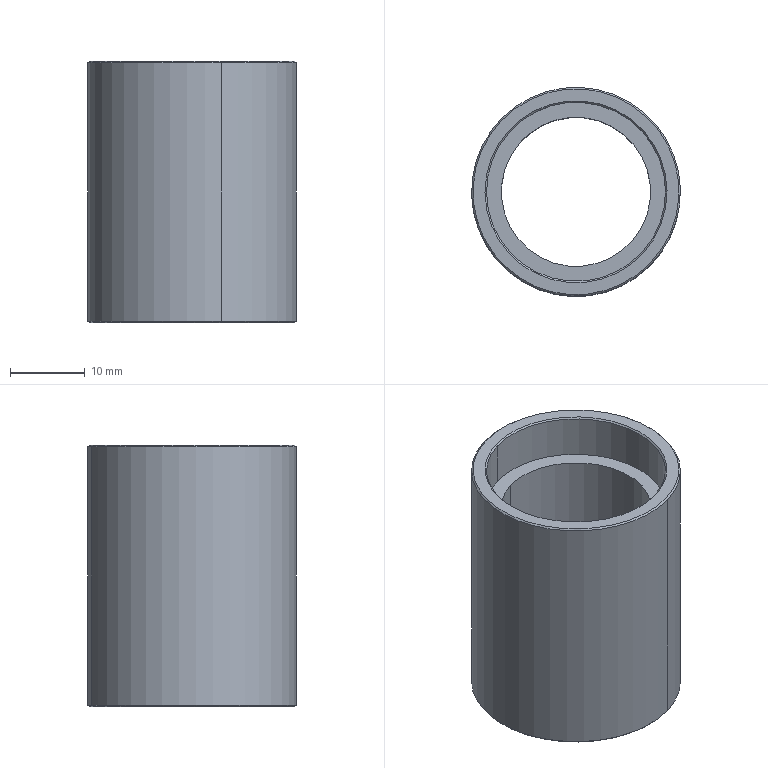Component | SolidWorks | GluePaperFeedingPressureRollerAssembly-1_YX-04-112GluePaperFeedingBearingFixingSleeve-1 | 1 solid | 20 faces | box 28 x 28 x 35 mm | volume 8890 mm3 | cylinder 8 | cone 8 | plane 4 | commonest cylinder face diameters 24 x4 20 x2 28 x2 | material 45#Steel
build123d program:
from build123d import *


with BuildPart() as part:
    # Sketch1 → Revolve1 (revolve)
    with BuildSketch(Plane.XY, mode=Mode.PRIVATE) as revolve1_sk:
        Polygon((-11.5, 12), (-11.5, 10), (11.5, 10), (11.5, 12), (17.3, 12), (17.5, 12.2), (17.5, 13.8), (17.3, 14), (-17.3, 14), (-17.5, 13.8), (-17.5, 12.2), (-17.3, 12), align=None)
    revolve(revolve1_sk.sketch.rotate(Axis((-17.5, 0, 0), (1, 0, 0)), 270), axis=Axis((-17.5, 0, 0), (1, 0, 0)))


solid = part.part

# Placed as in the assembly
solid = solid.moved(Location((-23.397, 0.262, 136.5), (0, 90, 0)))
STEP:
#1=COLOUR_RGB('',0.7922,0.8196,0.9333);
#2=FILL_AREA_STYLE_COLOUR('',#1);
#3=FILL_AREA_STYLE('',(#2));
#4=SURFACE_STYLE_FILL_AREA(#3);
#5=SURFACE_SIDE_STYLE('',(#4));
#6=SURFACE_STYLE_USAGE(.BOTH.,#5);
#7=PRESENTATION_STYLE_ASSIGNMENT((#6));
#8=CARTESIAN_POINT('',(-0.81,-0.3674,5.827));
#9=VERTEX_POINT('',#8);
#10=CARTESIAN_POINT('',(-1.032,0.388,5.827));
#11=VERTEX_POINT('',#10);
#12=CARTESIAN_POINT('',(-0.9212,0.01031,5.827));
#13=DIRECTION('',(-0.,0.,-1.));
#14=DIRECTION('',(-0.2824,0.9593,0.));
#15=AXIS2_PLACEMENT_3D('',#12,#13,#14);
#16=CIRCLE('',#15,0.3937);
#17=EDGE_CURVE('',#9,#11,#16,.T.);
#18=ORIENTED_EDGE('',*,*,#17,.F.);
#19=CARTESIAN_POINT('',(-0.81,-0.3674,4.921));
#20=VERTEX_POINT('',#19);
#21=CARTESIAN_POINT('',(-0.81,-0.3674,6.063));
#22=DIRECTION('',(-0.,0.,-1.));
#23=VECTOR('',#22,39.37);
#24=LINE('',#21,#23);
#25=EDGE_CURVE('',#9,#20,#24,.T.);
#26=ORIENTED_EDGE('',*,*,#25,.T.);
#27=CARTESIAN_POINT('',(-1.032,0.388,4.921));
#28=VERTEX_POINT('',#27);
#29=CARTESIAN_POINT('',(-0.9212,0.01031,4.921));
#30=DIRECTION('',(-0.,0.,-1.));
#31=DIRECTION('',(-0.2824,0.9593,0.));
#32=AXIS2_PLACEMENT_3D('',#29,#30,#31);
#33=CIRCLE('',#32,0.3937);
#34=EDGE_CURVE('',#20,#28,#33,.T.);
#35=ORIENTED_EDGE('',*,*,#34,.T.);
#36=CARTESIAN_POINT('',(-1.032,0.388,6.063));
#37=DIRECTION('',(-0.,0.,-1.));
#38=VECTOR('',#37,39.37);
#39=LINE('',#36,#38);
#40=EDGE_CURVE('',#11,#28,#39,.T.);
#41=ORIENTED_EDGE('',*,*,#40,.F.);
#42=EDGE_LOOP('',(#18,#26,#35,#41));
#43=FACE_OUTER_BOUND('',#42,.T.);
#44=CARTESIAN_POINT('',(-0.9212,0.01031,6.063));
#45=DIRECTION('',(-0.,0.,-1.));
#46=DIRECTION('',(-0.2824,0.9593,0.));
#47=AXIS2_PLACEMENT_3D('',#44,#45,#46);
#48=CYLINDRICAL_SURFACE('',#47,0.3937);
#49=ADVANCED_FACE('',(#43),#48,.F.);
#50=CARTESIAN_POINT('',(-0.7877,-0.4429,4.921));
#51=VERTEX_POINT('',#50);
#52=CARTESIAN_POINT('',(-1.055,0.4635,4.921));
#53=VERTEX_POINT('',#52);
#54=CARTESIAN_POINT('',(-0.9212,0.01031,4.921));
#55=DIRECTION('',(-0.,0.,-1.));
#56=DIRECTION('',(-0.2824,0.9593,0.));
#57=AXIS2_PLACEMENT_3D('',#54,#55,#56);
#58=CIRCLE('',#57,0.4724);
#59=EDGE_CURVE('',#51,#53,#58,.T.);
#60=ORIENTED_EDGE('',*,*,#59,.F.);
#61=CARTESIAN_POINT('',(-0.7877,-0.4429,4.693));
#62=VERTEX_POINT('',#61);
#63=CARTESIAN_POINT('',(-0.7877,-0.4429,6.063));
#64=DIRECTION('',(-0.,0.,-1.));
#65=VECTOR('',#64,39.37);
#66=LINE('',#63,#65);
#67=EDGE_CURVE('',#51,#62,#66,.T.);
#68=ORIENTED_EDGE('',*,*,#67,.T.);
#69=CARTESIAN_POINT('',(-1.055,0.4635,4.693));
#70=VERTEX_POINT('',#69);
#71=CARTESIAN_POINT('',(-0.9212,0.01031,4.693));
#72=DIRECTION('',(-0.,0.,-1.));
#73=DIRECTION('',(-0.2824,0.9593,0.));
#74=AXIS2_PLACEMENT_3D('',#71,#72,#73);
#75=CIRCLE('',#74,0.4724);
#76=EDGE_CURVE('',#62,#70,#75,.T.);
#77=ORIENTED_EDGE('',*,*,#76,.T.);
#78=CARTESIAN_POINT('',(-1.055,0.4635,6.063));
#79=DIRECTION('',(-0.,0.,-1.));
#80=VECTOR('',#79,39.37);
#81=LINE('',#78,#80);
#82=EDGE_CURVE('',#53,#70,#81,.T.);
#83=ORIENTED_EDGE('',*,*,#82,.F.);
#84=EDGE_LOOP('',(#60,#68,#77,#83));
#85=FACE_OUTER_BOUND('',#84,.T.);
#86=CARTESIAN_POINT('',(-0.9212,0.01031,6.063));
#87=DIRECTION('',(-0.,0.,-1.));
#88=DIRECTION('',(-0.2824,0.9593,0.));
#89=AXIS2_PLACEMENT_3D('',#86,#87,#88);
#90=CYLINDRICAL_SURFACE('',#89,0.4724);
#91=ADVANCED_FACE('',(#85),#90,.F.);
#92=ORIENTED_EDGE('',*,*,#76,.F.);
#93=CARTESIAN_POINT('',(-0.7855,-0.4505,4.685));
#94=VERTEX_POINT('',#93);
#95=CARTESIAN_POINT('',(-0.7877,-0.4429,4.693));
#96=DIRECTION('',(0.1997,-0.6783,-0.7071));
#97=VECTOR('',#96,39.37);
#98=LINE('',#95,#97);
#99=EDGE_CURVE('',#62,#94,#98,.T.);
#100=ORIENTED_EDGE('',*,*,#99,.T.);
#101=CARTESIAN_POINT('',(-1.057,0.4711,4.685));
#102=VERTEX_POINT('',#101);
#103=CARTESIAN_POINT('',(-0.9212,0.01031,4.685));
#104=DIRECTION('',(-0.,0.,-1.));
#105=DIRECTION('',(-0.2824,0.9593,0.));
#106=AXIS2_PLACEMENT_3D('',#103,#104,#105);
#107=CIRCLE('',#106,0.4803);
#108=EDGE_CURVE('',#94,#102,#107,.T.);
#109=ORIENTED_EDGE('',*,*,#108,.T.);
#110=CARTESIAN_POINT('',(-1.055,0.4635,4.693));
#111=DIRECTION('',(-0.1997,0.6783,-0.7071));
#112=VECTOR('',#111,39.37);
#113=LINE('',#110,#112);
#114=EDGE_CURVE('',#70,#102,#113,.T.);
#115=ORIENTED_EDGE('',*,*,#114,.F.);
#116=EDGE_LOOP('',(#92,#100,#109,#115));
#117=FACE_OUTER_BOUND('',#116,.T.);
#118=CARTESIAN_POINT('',(-0.9212,0.01031,4.693));
#119=DIRECTION('',(-0.,0.,-1.));
#120=DIRECTION('',(-0.2824,0.9593,0.));
#121=AXIS2_PLACEMENT_3D('',#118,#119,#120);
#122=CONICAL_SURFACE('',#121,0.4724,0.7854);
#123=ADVANCED_FACE('',(#117),#122,.F.);
#124=CARTESIAN_POINT('',(-1.075,0.5315,4.685));
#125=VERTEX_POINT('',#124);
#126=CARTESIAN_POINT('',(-0.7677,-0.5109,4.685));
#127=VERTEX_POINT('',#126);
#128=CARTESIAN_POINT('',(-0.9212,0.01031,4.685));
#129=DIRECTION('',(-0.,0.,-1.));
#130=DIRECTION('',(-0.2824,0.9593,0.));
#131=AXIS2_PLACEMENT_3D('',#128,#129,#130);
#132=CIRCLE('',#131,0.5433);
#133=EDGE_CURVE('',#125,#127,#132,.T.);
#134=ORIENTED_EDGE('',*,*,#133,.F.);
#135=CARTESIAN_POINT('',(-1.077,0.5391,4.693));
#136=VERTEX_POINT('',#135);
#137=CARTESIAN_POINT('',(-1.075,0.5315,4.685));
#138=DIRECTION('',(-0.1997,0.6783,0.7071));
#139=VECTOR('',#138,39.37);
#140=LINE('',#137,#139);
#141=EDGE_CURVE('',#125,#136,#140,.T.);
#142=ORIENTED_EDGE('',*,*,#141,.T.);
#143=CARTESIAN_POINT('',(-0.7655,-0.5184,4.693));
#144=VERTEX_POINT('',#143);
#145=CARTESIAN_POINT('',(-0.9212,0.01031,4.693));
#146=DIRECTION('',(-0.,0.,-1.));
#147=DIRECTION('',(-0.2824,0.9593,0.));
#148=AXIS2_PLACEMENT_3D('',#145,#146,#147);
#149=CIRCLE('',#148,0.5512);
#150=EDGE_CURVE('',#136,#144,#149,.T.);
#151=ORIENTED_EDGE('',*,*,#150,.T.);
#152=CARTESIAN_POINT('',(-0.7677,-0.5109,4.685));
#153=DIRECTION('',(0.1997,-0.6783,0.7071));
#154=VECTOR('',#153,39.37);
#155=LINE('',#152,#154);
#156=EDGE_CURVE('',#127,#144,#155,.T.);
#157=ORIENTED_EDGE('',*,*,#156,.F.);
#158=EDGE_LOOP('',(#134,#142,#151,#157));
#159=FACE_OUTER_BOUND('',#158,.T.);
#160=CARTESIAN_POINT('',(-0.9212,0.01031,4.685));
#161=DIRECTION('',(0.,-0.,1.));
#162=DIRECTION('',(0.2824,-0.9593,0.));
#163=AXIS2_PLACEMENT_3D('',#160,#161,#162);
#164=CONICAL_SURFACE('',#163,0.5433,0.7854);
#165=ADVANCED_FACE('',(#159),#164,.T.);
#166=CARTESIAN_POINT('',(-1.077,0.5391,6.055));
#167=VERTEX_POINT('',#166);
#168=CARTESIAN_POINT('',(-0.7655,-0.5184,6.055));
#169=VERTEX_POINT('',#168);
#170=CARTESIAN_POINT('',(-0.9212,0.01031,6.055));
#171=DIRECTION('',(-0.,0.,-1.));
#172=DIRECTION('',(-0.2824,0.9593,0.));
#173=AXIS2_PLACEMENT_3D('',#170,#171,#172);
#174=CIRCLE('',#173,0.5512);
#175=EDGE_CURVE('',#167,#169,#174,.T.);
#176=ORIENTED_EDGE('',*,*,#175,.T.);
#177=CARTESIAN_POINT('',(-0.7655,-0.5184,6.063));
#178=DIRECTION('',(-0.,0.,-1.));
#179=VECTOR('',#178,39.37);
#180=LINE('',#177,#179);
#181=EDGE_CURVE('',#169,#144,#180,.T.);
#182=ORIENTED_EDGE('',*,*,#181,.T.);
#183=ORIENTED_EDGE('',*,*,#150,.F.);
#184=CARTESIAN_POINT('',(-1.077,0.5391,6.063));
#185=DIRECTION('',(-0.,0.,-1.));
#186=VECTOR('',#185,39.37);
#187=LINE('',#184,#186);
#188=EDGE_CURVE('',#167,#136,#187,.T.);
#189=ORIENTED_EDGE('',*,*,#188,.F.);
#190=EDGE_LOOP('',(#176,#182,#183,#189));
#191=FACE_OUTER_BOUND('',#190,.T.);
#192=CARTESIAN_POINT('',(-0.9212,0.01031,6.063));
#193=DIRECTION('',(-0.,0.,-1.));
#194=DIRECTION('',(-0.2824,0.9593,0.));
#195=AXIS2_PLACEMENT_3D('',#192,#193,#194);
#196=CYLINDRICAL_SURFACE('',#195,0.5512);
#197=ADVANCED_FACE('',(#191),#196,.T.);
#198=CARTESIAN_POINT('',(-1.075,0.5315,6.063));
#199=VERTEX_POINT('',#198);
#200=CARTESIAN_POINT('',(-0.7677,-0.5109,6.063));
#201=VERTEX_POINT('',#200);
#202=CARTESIAN_POINT('',(-0.9212,0.01031,6.063));
#203=DIRECTION('',(-0.,0.,-1.));
#204=DIRECTION('',(-0.2824,0.9593,0.));
#205=AXIS2_PLACEMENT_3D('',#202,#203,#204);
#206=CIRCLE('',#205,0.5433);
#207=EDGE_CURVE('',#199,#201,#206,.T.);
#208=ORIENTED_EDGE('',*,*,#207,.T.);
#209=CARTESIAN_POINT('',(-0.7655,-0.5184,6.055));
#210=DIRECTION('',(0.1997,-0.6783,-0.7071));
#211=VECTOR('',#210,39.37);
#212=LINE('',#209,#211);
#213=EDGE_CURVE('',#201,#169,#212,.T.);
#214=ORIENTED_EDGE('',*,*,#213,.T.);
#215=ORIENTED_EDGE('',*,*,#175,.F.);
#216=CARTESIAN_POINT('',(-1.077,0.5391,6.055));
#217=DIRECTION('',(-0.1997,0.6783,-0.7071));
#218=VECTOR('',#217,39.37);
#219=LINE('',#216,#218);
#220=EDGE_CURVE('',#199,#167,#219,.T.);
#221=ORIENTED_EDGE('',*,*,#220,.F.);
#222=EDGE_LOOP('',(#208,#214,#215,#221));
#223=FACE_OUTER_BOUND('',#222,.T.);
#224=CARTESIAN_POINT('',(-0.9212,0.01031,6.055));
#225=DIRECTION('',(-0.,0.,-1.));
#226=DIRECTION('',(-0.2824,0.9593,0.));
#227=AXIS2_PLACEMENT_3D('',#224,#225,#226);
#228=CONICAL_SURFACE('',#227,0.5512,0.7854);
#229=ADVANCED_FACE('',(#223),#228,.T.);
#230=CARTESIAN_POINT('',(-0.7877,-0.4429,6.055));
#231=VERTEX_POINT('',#230);
#232=CARTESIAN_POINT('',(-1.055,0.4635,6.055));
#233=VERTEX_POINT('',#232);
#234=CARTESIAN_POINT('',(-0.9212,0.01031,6.055));
#235=DIRECTION('',(-0.,0.,-1.));
#236=DIRECTION('',(-0.2824,0.9593,0.));
#237=AXIS2_PLACEMENT_3D('',#234,#235,#236);
#238=CIRCLE('',#237,0.4724);
#239=EDGE_CURVE('',#231,#233,#238,.T.);
#240=ORIENTED_EDGE('',*,*,#239,.T.);
#241=CARTESIAN_POINT('',(-1.057,0.4711,6.063));
#242=VERTEX_POINT('',#241);
#243=CARTESIAN_POINT('',(-1.057,0.4711,6.063));
#244=DIRECTION('',(-0.1997,0.6783,0.7071));
#245=VECTOR('',#244,39.37);
#246=LINE('',#243,#245);
#247=EDGE_CURVE('',#233,#242,#246,.T.);
#248=ORIENTED_EDGE('',*,*,#247,.T.);
#249=CARTESIAN_POINT('',(-0.7855,-0.4505,6.063));
#250=VERTEX_POINT('',#249);
#251=CARTESIAN_POINT('',(-0.9212,0.01031,6.063));
#252=DIRECTION('',(-0.,0.,-1.));
#253=DIRECTION('',(-0.2824,0.9593,0.));
#254=AXIS2_PLACEMENT_3D('',#251,#252,#253);
#255=CIRCLE('',#254,0.4803);
#256=EDGE_CURVE('',#250,#242,#255,.T.);
#257=ORIENTED_EDGE('',*,*,#256,.F.);
#258=CARTESIAN_POINT('',(-0.7855,-0.4505,6.063));
#259=DIRECTION('',(0.1997,-0.6783,0.7071));
#260=VECTOR('',#259,39.37);
#261=LINE('',#258,#260);
#262=EDGE_CURVE('',#231,#250,#261,.T.);
#263=ORIENTED_EDGE('',*,*,#262,.F.);
#264=EDGE_LOOP('',(#240,#248,#257,#263));
#265=FACE_OUTER_BOUND('',#264,.T.);
#266=CARTESIAN_POINT('',(-0.9212,0.01031,6.063));
#267=DIRECTION('',(0.,-0.,1.));
#268=DIRECTION('',(0.2824,-0.9593,0.));
#269=AXIS2_PLACEMENT_3D('',#266,#267,#268);
#270=CONICAL_SURFACE('',#269,0.4803,0.7854);
#271=ADVANCED_FACE('',(#265),#270,.F.);
#272=ORIENTED_EDGE('',*,*,#239,.F.);
#273=CARTESIAN_POINT('',(-0.7877,-0.4429,5.827));
#274=VERTEX_POINT('',#273);
#275=CARTESIAN_POINT('',(-0.7877,-0.4429,6.063));
#276=DIRECTION('',(-0.,0.,-1.));
#277=VECTOR('',#276,39.37);
#278=LINE('',#275,#277);
#279=EDGE_CURVE('',#231,#274,#278,.T.);
#280=ORIENTED_EDGE('',*,*,#279,.T.);
#281=CARTESIAN_POINT('',(-1.055,0.4635,5.827));
#282=VERTEX_POINT('',#281);
#283=CARTESIAN_POINT('',(-0.9212,0.01031,5.827));
#284=DIRECTION('',(-0.,0.,-1.));
#285=DIRECTION('',(-0.2824,0.9593,0.));
#286=AXIS2_PLACEMENT_3D('',#283,#284,#285);
#287=CIRCLE('',#286,0.4724);
#288=EDGE_CURVE('',#274,#282,#287,.T.);
#289=ORIENTED_EDGE('',*,*,#288,.T.);
#290=CARTESIAN_POINT('',(-1.055,0.4635,6.063));
#291=DIRECTION('',(-0.,0.,-1.));
#292=VECTOR('',#291,39.37);
#293=LINE('',#290,#292);
#294=EDGE_CURVE('',#233,#282,#293,.T.);
#295=ORIENTED_EDGE('',*,*,#294,.F.);
#296=EDGE_LOOP('',(#272,#280,#289,#295));
#297=FACE_OUTER_BOUND('',#296,.T.);
#298=CARTESIAN_POINT('',(-0.9212,0.01031,6.063));
#299=DIRECTION('',(-0.,0.,-1.));
#300=DIRECTION('',(-0.2824,0.9593,0.));
#301=AXIS2_PLACEMENT_3D('',#298,#299,#300);
#302=CYLINDRICAL_SURFACE('',#301,0.4724);
#303=ADVANCED_FACE('',(#297),#302,.F.);
#304=ORIENTED_EDGE('',*,*,#279,.F.);
#305=CARTESIAN_POINT('',(-0.9212,0.01031,6.055));
#306=DIRECTION('',(-0.,0.,-1.));
#307=DIRECTION('',(-0.2824,0.9593,0.));
#308=AXIS2_PLACEMENT_3D('',#305,#306,#307);
#309=CIRCLE('',#308,0.4724);
#310=EDGE_CURVE('',#233,#231,#309,.T.);
#311=ORIENTED_EDGE('',*,*,#310,.F.);
#312=ORIENTED_EDGE('',*,*,#294,.T.);
#313=CARTESIAN_POINT('',(-0.9212,0.01031,5.827));
#314=DIRECTION('',(-0.,0.,-1.));
#315=DIRECTION('',(-0.2824,0.9593,0.));
#316=AXIS2_PLACEMENT_3D('',#313,#314,#315);
#317=CIRCLE('',#316,0.4724);
#318=EDGE_CURVE('',#282,#274,#317,.T.);
#319=ORIENTED_EDGE('',*,*,#318,.T.);
#320=EDGE_LOOP('',(#304,#311,#312,#319));
#321=FACE_OUTER_BOUND('',#320,.T.);
#322=CARTESIAN_POINT('',(-0.9212,0.01031,6.063));
#323=DIRECTION('',(-0.,0.,-1.));
#324=DIRECTION('',(-0.2824,0.9593,0.));
#325=AXIS2_PLACEMENT_3D('',#322,#323,#324);
#326=CYLINDRICAL_SURFACE('',#325,0.4724);
#327=ADVANCED_FACE('',(#321),#326,.F.);
#328=ORIENTED_EDGE('',*,*,#247,.F.);
#329=ORIENTED_EDGE('',*,*,#310,.T.);
#330=ORIENTED_EDGE('',*,*,#262,.T.);
#331=CARTESIAN_POINT('',(-0.9212,0.01031,6.063));
#332=DIRECTION('',(-0.,0.,-1.));
#333=DIRECTION('',(-0.2824,0.9593,0.));
#334=AXIS2_PLACEMENT_3D('',#331,#332,#333);
#335=CIRCLE('',#334,0.4803);
#336=EDGE_CURVE('',#242,#250,#335,.T.);
#337=ORIENTED_EDGE('',*,*,#336,.F.);
#338=EDGE_LOOP('',(#328,#329,#330,#337));
#339=FACE_OUTER_BOUND('',#338,.T.);
#340=CARTESIAN_POINT('',(-0.9212,0.01031,6.063));
#341=DIRECTION('',(0.,-0.,1.));
#342=DIRECTION('',(0.2824,-0.9593,0.));
#343=AXIS2_PLACEMENT_3D('',#340,#341,#342);
#344=CONICAL_SURFACE('',#343,0.4803,0.7854);
#345=ADVANCED_FACE('',(#339),#344,.F.);
#346=ORIENTED_EDGE('',*,*,#256,.T.);
#347=ORIENTED_EDGE('',*,*,#336,.T.);
#348=EDGE_LOOP('',(#346,#347));
#349=FACE_BOUND('',#348,.T.);
#350=ORIENTED_EDGE('',*,*,#207,.F.);
#351=CARTESIAN_POINT('',(-0.9212,0.01031,6.063));
#352=DIRECTION('',(-0.,0.,-1.));
#353=DIRECTION('',(-0.2824,0.9593,0.));
#354=AXIS2_PLACEMENT_3D('',#351,#352,#353);
#355=CIRCLE('',#354,0.5433);
#356=EDGE_CURVE('',#201,#199,#355,.T.);
#357=ORIENTED_EDGE('',*,*,#356,.F.);
#358=EDGE_LOOP('',(#350,#357));
#359=FACE_OUTER_BOUND('',#358,.T.);
#360=CARTESIAN_POINT('',(-0.4,0.1637,6.063));
#361=DIRECTION('',(0.,-0.,1.));
#362=DIRECTION('',(0.2824,-0.9593,-0.));
#363=AXIS2_PLACEMENT_3D('',#360,#361,#362);
#364=PLANE('',#363);
#365=ADVANCED_FACE('',(#349,#359),#364,.T.);
#366=ORIENTED_EDGE('',*,*,#213,.F.);
#367=ORIENTED_EDGE('',*,*,#356,.T.);
#368=ORIENTED_EDGE('',*,*,#220,.T.);
#369=CARTESIAN_POINT('',(-0.9212,0.01031,6.055));
#370=DIRECTION('',(-0.,0.,-1.));
#371=DIRECTION('',(-0.2824,0.9593,0.));
#372=AXIS2_PLACEMENT_3D('',#369,#370,#371);
#373=CIRCLE('',#372,0.5512);
#374=EDGE_CURVE('',#169,#167,#373,.T.);
#375=ORIENTED_EDGE('',*,*,#374,.F.);
#376=EDGE_LOOP('',(#366,#367,#368,#375));
#377=FACE_OUTER_BOUND('',#376,.T.);
#378=CARTESIAN_POINT('',(-0.9212,0.01031,6.055));
#379=DIRECTION('',(-0.,0.,-1.));
#380=DIRECTION('',(-0.2824,0.9593,0.));
#381=AXIS2_PLACEMENT_3D('',#378,#379,#380);
#382=CONICAL_SURFACE('',#381,0.5512,0.7854);
#383=ADVANCED_FACE('',(#377),#382,.T.);
#384=ORIENTED_EDGE('',*,*,#181,.F.);
#385=ORIENTED_EDGE('',*,*,#374,.T.);
#386=ORIENTED_EDGE('',*,*,#188,.T.);
#387=CARTESIAN_POINT('',(-0.9212,0.01031,4.693));
#388=DIRECTION('',(-0.,0.,-1.));
#389=DIRECTION('',(-0.2824,0.9593,0.));
#390=AXIS2_PLACEMENT_3D('',#387,#388,#389);
#391=CIRCLE('',#390,0.5512);
#392=EDGE_CURVE('',#144,#136,#391,.T.);
#393=ORIENTED_EDGE('',*,*,#392,.F.);
#394=EDGE_LOOP('',(#384,#385,#386,#393));
#395=FACE_OUTER_BOUND('',#394,.T.);
#396=CARTESIAN_POINT('',(-0.9212,0.01031,6.063));
#397=DIRECTION('',(-0.,0.,-1.));
#398=DIRECTION('',(-0.2824,0.9593,0.));
#399=AXIS2_PLACEMENT_3D('',#396,#397,#398);
#400=CYLINDRICAL_SURFACE('',#399,0.5512);
#401=ADVANCED_FACE('',(#395),#400,.T.);
#402=ORIENTED_EDGE('',*,*,#141,.F.);
#403=CARTESIAN_POINT('',(-0.9212,0.01031,4.685));
#404=DIRECTION('',(-0.,0.,-1.));
#405=DIRECTION('',(-0.2824,0.9593,0.));
#406=AXIS2_PLACEMENT_3D('',#403,#404,#405);
#407=CIRCLE('',#406,0.5433);
#408=EDGE_CURVE('',#127,#125,#407,.T.);
#409=ORIENTED_EDGE('',*,*,#408,.F.);
#410=ORIENTED_EDGE('',*,*,#156,.T.);
#411=ORIENTED_EDGE('',*,*,#392,.T.);
#412=EDGE_LOOP('',(#402,#409,#410,#411));
#413=FACE_OUTER_BOUND('',#412,.T.);
#414=CARTESIAN_POINT('',(-0.9212,0.01031,4.685));
#415=DIRECTION('',(0.,-0.,1.));
#416=DIRECTION('',(0.2824,-0.9593,0.));
#417=AXIS2_PLACEMENT_3D('',#414,#415,#416);
#418=CONICAL_SURFACE('',#417,0.5433,0.7854);
#419=ADVANCED_FACE('',(#413),#418,.T.);
#420=ORIENTED_EDGE('',*,*,#408,.T.);
#421=ORIENTED_EDGE('',*,*,#133,.T.);
#422=EDGE_LOOP('',(#420,#421));
#423=FACE_OUTER_BOUND('',#422,.T.);
#424=CARTESIAN_POINT('',(-0.9212,0.01031,4.685));
#425=DIRECTION('',(-0.,0.,-1.));
#426=DIRECTION('',(-0.2824,0.9593,0.));
#427=AXIS2_PLACEMENT_3D('',#424,#425,#426);
#428=CIRCLE('',#427,0.4803);
#429=EDGE_CURVE('',#102,#94,#428,.T.);
#430=ORIENTED_EDGE('',*,*,#429,.F.);
#431=ORIENTED_EDGE('',*,*,#108,.F.);
#432=EDGE_LOOP('',(#430,#431));
#433=FACE_BOUND('',#432,.T.);
#434=CARTESIAN_POINT('',(-0.4604,0.146,4.685));
#435=DIRECTION('',(-0.,0.,-1.));
#436=DIRECTION('',(-0.2824,0.9593,0.));
#437=AXIS2_PLACEMENT_3D('',#434,#435,#436);
#438=PLANE('',#437);
#439=ADVANCED_FACE('',(#423,#433),#438,.T.);
#440=ORIENTED_EDGE('',*,*,#99,.F.);
#441=CARTESIAN_POINT('',(-0.9212,0.01031,4.693));
#442=DIRECTION('',(-0.,0.,-1.));
#443=DIRECTION('',(-0.2824,0.9593,0.));
#444=AXIS2_PLACEMENT_3D('',#441,#442,#443);
#445=CIRCLE('',#444,0.4724);
#446=EDGE_CURVE('',#70,#62,#445,.T.);
#447=ORIENTED_EDGE('',*,*,#446,.F.);
#448=ORIENTED_EDGE('',*,*,#114,.T.);
#449=ORIENTED_EDGE('',*,*,#429,.T.);
#450=EDGE_LOOP('',(#440,#447,#448,#449));
#451=FACE_OUTER_BOUND('',#450,.T.);
#452=CARTESIAN_POINT('',(-0.9212,0.01031,4.693));
#453=DIRECTION('',(-0.,0.,-1.));
#454=DIRECTION('',(-0.2824,0.9593,0.));
#455=AXIS2_PLACEMENT_3D('',#452,#453,#454);
#456=CONICAL_SURFACE('',#455,0.4724,0.7854);
#457=ADVANCED_FACE('',(#451),#456,.F.);
#458=ORIENTED_EDGE('',*,*,#67,.F.);
#459=CARTESIAN_POINT('',(-0.9212,0.01031,4.921));
#460=DIRECTION('',(-0.,0.,-1.));
#461=DIRECTION('',(-0.2824,0.9593,0.));
#462=AXIS2_PLACEMENT_3D('',#459,#460,#461);
#463=CIRCLE('',#462,0.4724);
#464=EDGE_CURVE('',#53,#51,#463,.T.);
#465=ORIENTED_EDGE('',*,*,#464,.F.);
#466=ORIENTED_EDGE('',*,*,#82,.T.);
#467=ORIENTED_EDGE('',*,*,#446,.T.);
#468=EDGE_LOOP('',(#458,#465,#466,#467));
#469=FACE_OUTER_BOUND('',#468,.T.);
#470=CARTESIAN_POINT('',(-0.9212,0.01031,6.063));
#471=DIRECTION('',(-0.,0.,-1.));
#472=DIRECTION('',(-0.2824,0.9593,0.));
#473=AXIS2_PLACEMENT_3D('',#470,#471,#472);
#474=CYLINDRICAL_SURFACE('',#473,0.4724);
#475=ADVANCED_FACE('',(#469),#474,.F.);
#476=ORIENTED_EDGE('',*,*,#464,.T.);
#477=ORIENTED_EDGE('',*,*,#59,.T.);
#478=EDGE_LOOP('',(#476,#477));
#479=FACE_OUTER_BOUND('',#478,.T.);
#480=CARTESIAN_POINT('',(-0.9212,0.01031,4.921));
#481=DIRECTION('',(-0.,0.,-1.));
#482=DIRECTION('',(-0.2824,0.9593,0.));
#483=AXIS2_PLACEMENT_3D('',#480,#481,#482);
#484=CIRCLE('',#483,0.3937);
#485=EDGE_CURVE('',#28,#20,#484,.T.);
#486=ORIENTED_EDGE('',*,*,#485,.F.);
#487=ORIENTED_EDGE('',*,*,#34,.F.);
#488=EDGE_LOOP('',(#486,#487));
#489=FACE_BOUND('',#488,.T.);
#490=CARTESIAN_POINT('',(-0.5435,0.1215,4.921));
#491=DIRECTION('',(-0.,0.,-1.));
#492=DIRECTION('',(-0.2824,0.9593,0.));
#493=AXIS2_PLACEMENT_3D('',#490,#491,#492);
#494=PLANE('',#493);
#495=ADVANCED_FACE('',(#479,#489),#494,.T.);
#496=ORIENTED_EDGE('',*,*,#25,.F.);
#497=CARTESIAN_POINT('',(-0.9212,0.01031,5.827));
#498=DIRECTION('',(-0.,0.,-1.));
#499=DIRECTION('',(-0.2824,0.9593,0.));
#500=AXIS2_PLACEMENT_3D('',#497,#498,#499);
#501=CIRCLE('',#500,0.3937);
#502=EDGE_CURVE('',#11,#9,#501,.T.);
#503=ORIENTED_EDGE('',*,*,#502,.F.);
#504=ORIENTED_EDGE('',*,*,#40,.T.);
#505=ORIENTED_EDGE('',*,*,#485,.T.);
#506=EDGE_LOOP('',(#496,#503,#504,#505));
#507=FACE_OUTER_BOUND('',#506,.T.);
#508=CARTESIAN_POINT('',(-0.9212,0.01031,6.063));
#509=DIRECTION('',(-0.,0.,-1.));
#510=DIRECTION('',(-0.2824,0.9593,0.));
#511=AXIS2_PLACEMENT_3D('',#508,#509,#510);
#512=CYLINDRICAL_SURFACE('',#511,0.3937);
#513=ADVANCED_FACE('',(#507),#512,.F.);
#514=ORIENTED_EDGE('',*,*,#502,.T.);
#515=ORIENTED_EDGE('',*,*,#17,.T.);
#516=EDGE_LOOP('',(#514,#515));
#517=FACE_BOUND('',#516,.T.);
#518=ORIENTED_EDGE('',*,*,#318,.F.);
#519=ORIENTED_EDGE('',*,*,#288,.F.);
#520=EDGE_LOOP('',(#518,#519));
#521=FACE_OUTER_BOUND('',#520,.T.);
#522=CARTESIAN_POINT('',(-0.4679,0.1437,5.827));
#523=DIRECTION('',(0.,-0.,1.));
#524=DIRECTION('',(0.2824,-0.9593,-0.));
#525=AXIS2_PLACEMENT_3D('',#522,#523,#524);
#526=PLANE('',#525);
#527=ADVANCED_FACE('',(#517,#521),#526,.T.);
#528=CLOSED_SHELL('',(#49,#91,#123,#165,#197,#229,#271,#303,#327,#345,#365,#383,#401,#419,#439,#457,#475,#495,#513,#527));
#529=MANIFOLD_SOLID_BREP('',#528);
#530=STYLED_ITEM('',(#7),#529);
#531=PRESENTATION_LAYER_ASSIGNMENT('','',(#530));
#532=(LENGTH_UNIT()NAMED_UNIT(*)SI_UNIT($,.METRE.));
#533=LENGTH_MEASURE_WITH_UNIT(LENGTH_MEASURE(0.0254),#532);
#534=DIMENSIONAL_EXPONENTS(1.,0.,0.,0.,0.,0.,0.);
#535=(CONVERSION_BASED_UNIT('',#533)LENGTH_UNIT()NAMED_UNIT(#534));
#536=UNCERTAINTY_MEASURE_WITH_UNIT(LENGTH_MEASURE(0.00001),#535,'','');
#537=(NAMED_UNIT(*)PLANE_ANGLE_UNIT()SI_UNIT($,.RADIAN.));
#538=(NAMED_UNIT(*)SI_UNIT($,.STERADIAN.)SOLID_ANGLE_UNIT());
#539=(GEOMETRIC_REPRESENTATION_CONTEXT(3)GLOBAL_UNCERTAINTY_ASSIGNED_CONTEXT((#536))GLOBAL_UNIT_ASSIGNED_CONTEXT((#535,#537,#538))REPRESENTATION_CONTEXT('',''));
#540=MECHANICAL_DESIGN_GEOMETRIC_PRESENTATION_REPRESENTATION('',(#530),#539);
#541=CARTESIAN_POINT('',(0.,0.,0.));
#542=DIRECTION('',(0.,0.,1.));
#543=DIRECTION('',(1.,0.,0.));
#544=AXIS2_PLACEMENT_3D('',#541,#542,#543);
#545=(LENGTH_UNIT()NAMED_UNIT(*)SI_UNIT($,.METRE.));
#546=LENGTH_MEASURE_WITH_UNIT(LENGTH_MEASURE(0.0254),#545);
#547=DIMENSIONAL_EXPONENTS(1.,0.,0.,0.,0.,0.,0.);
#548=(CONVERSION_BASED_UNIT('',#546)LENGTH_UNIT()NAMED_UNIT(#547));
#549=UNCERTAINTY_MEASURE_WITH_UNIT(LENGTH_MEASURE(0.00001),#548,'','');
#550=(NAMED_UNIT(*)PLANE_ANGLE_UNIT()SI_UNIT($,.RADIAN.));
#551=(NAMED_UNIT(*)SI_UNIT($,.STERADIAN.)SOLID_ANGLE_UNIT());
#552=(GEOMETRIC_REPRESENTATION_CONTEXT(3)GLOBAL_UNCERTAINTY_ASSIGNED_CONTEXT((#549))GLOBAL_UNIT_ASSIGNED_CONTEXT((#548,#550,#551))REPRESENTATION_CONTEXT('',''));
#553=ADVANCED_BREP_SHAPE_REPRESENTATION('',(#529,#544),#552);